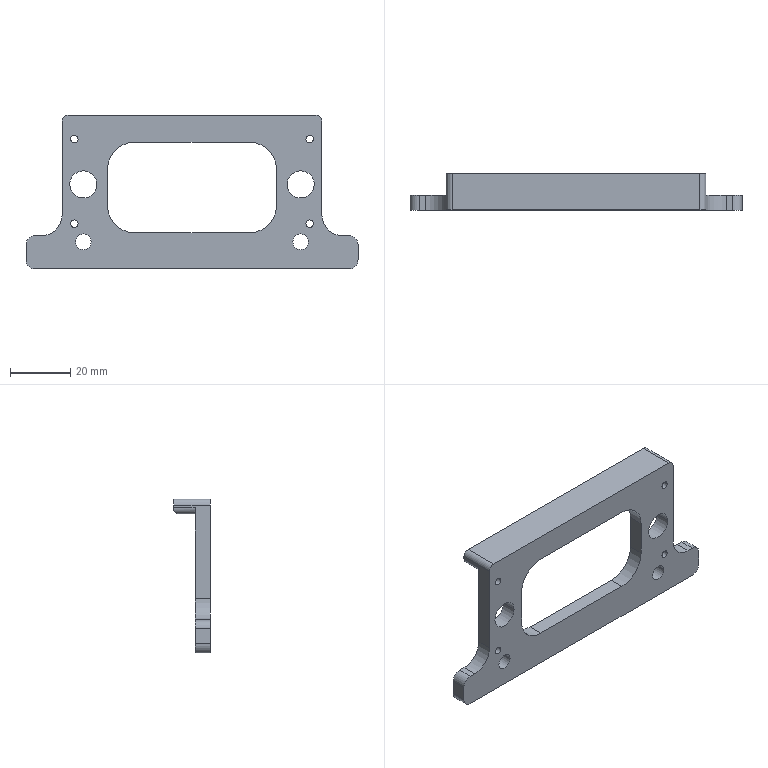CAM job | Mastercam | mm | 16 operations | part box 110 x 12 x 51
1. Facing | 24 - 100 平铣刀
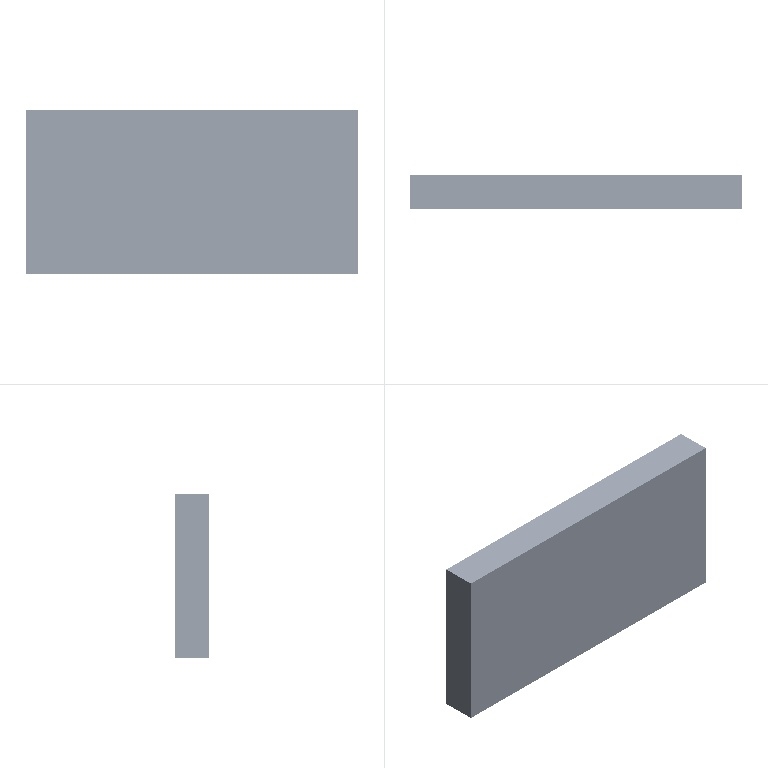2. 2D High Speed (2D Dynamic Mill) | 10 - 10 平铣刀
3. Contour (Ramp) | 10 - 10 平铣刀
4. Contour (2D) | 10 - 10 平铣刀
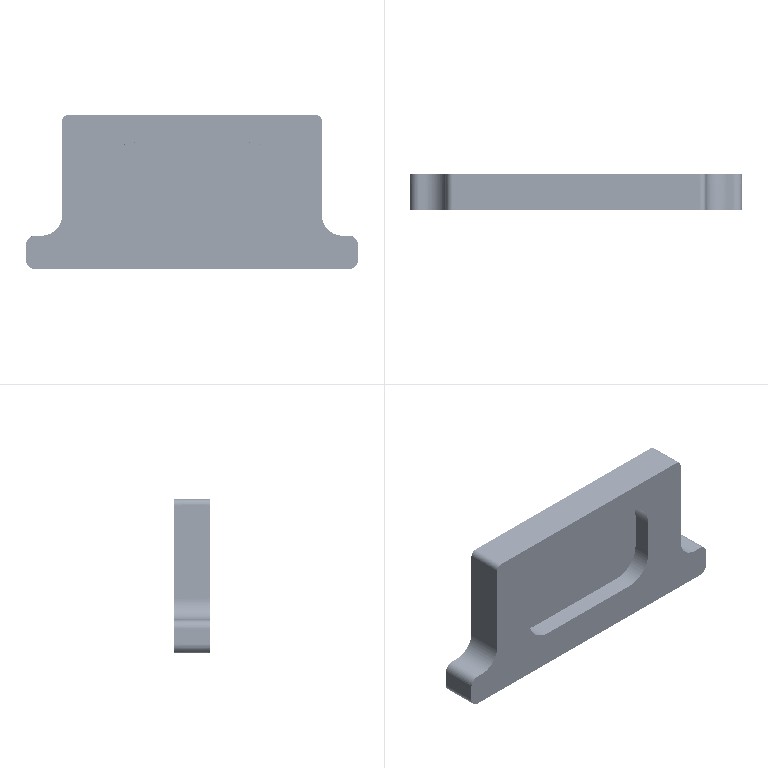5. Contour (2D) | 10 - 10 平铣刀
6. Contour (Ramp) | 6 - 6 平铣刀
7. Contour (2D) | 6 - 6 平铣刀
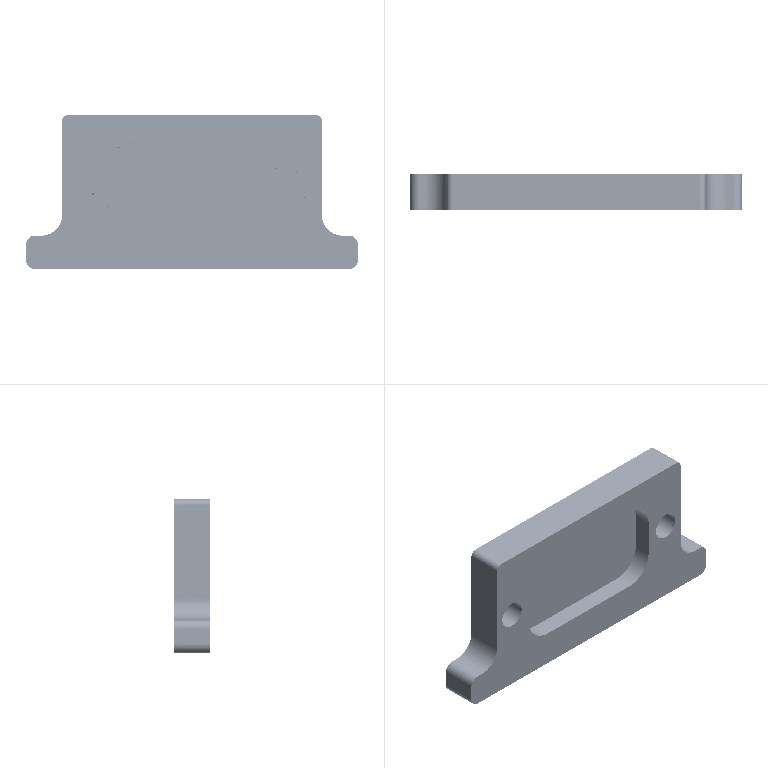8. Contour (2D chamfer) | 7 - 4 倒角刀
9. Facing | 24 - 100 平铣刀
10. Contour (Ramp) | 24 - 100 平铣刀
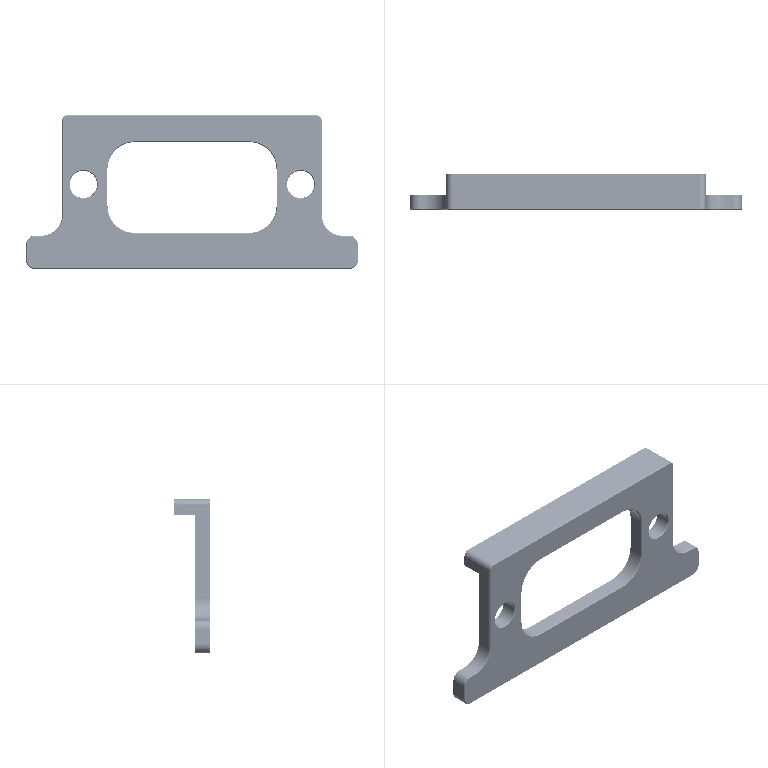11. Contour (2D) | 10 - 10 平铣刀
12. Contour (2D) | 10 - 10 平铣刀
13. Drill/Counterbore | 7 - 4 倒角刀
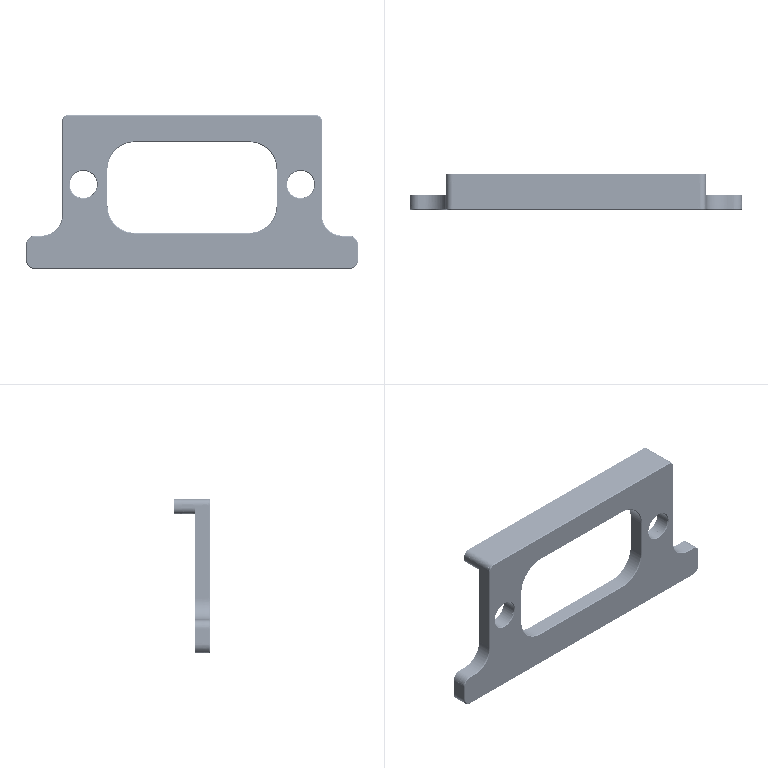14. Contour (2D chamfer) | 7 - 4 倒角刀
15. Contour (2D chamfer) | 7 - 4 倒角刀
16. Contour (2D chamfer) | 7 - 4 倒角刀